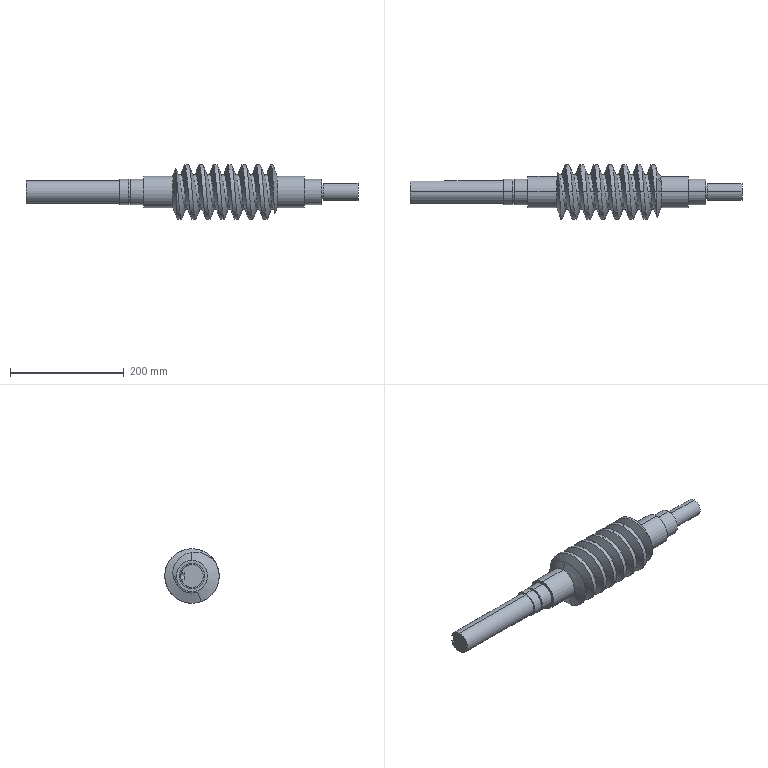Component | SolidWorks | 8Worm-1 | 1 solid | 68 faces | volume 1512466 mm3 | cylinder 50 | plane 12 | cone 4 | spline 2 | commonest cylinder face diameters 60 x16 96 x15 45 x6 55 x4 30 x2 26 x2 41 x2 40 x2